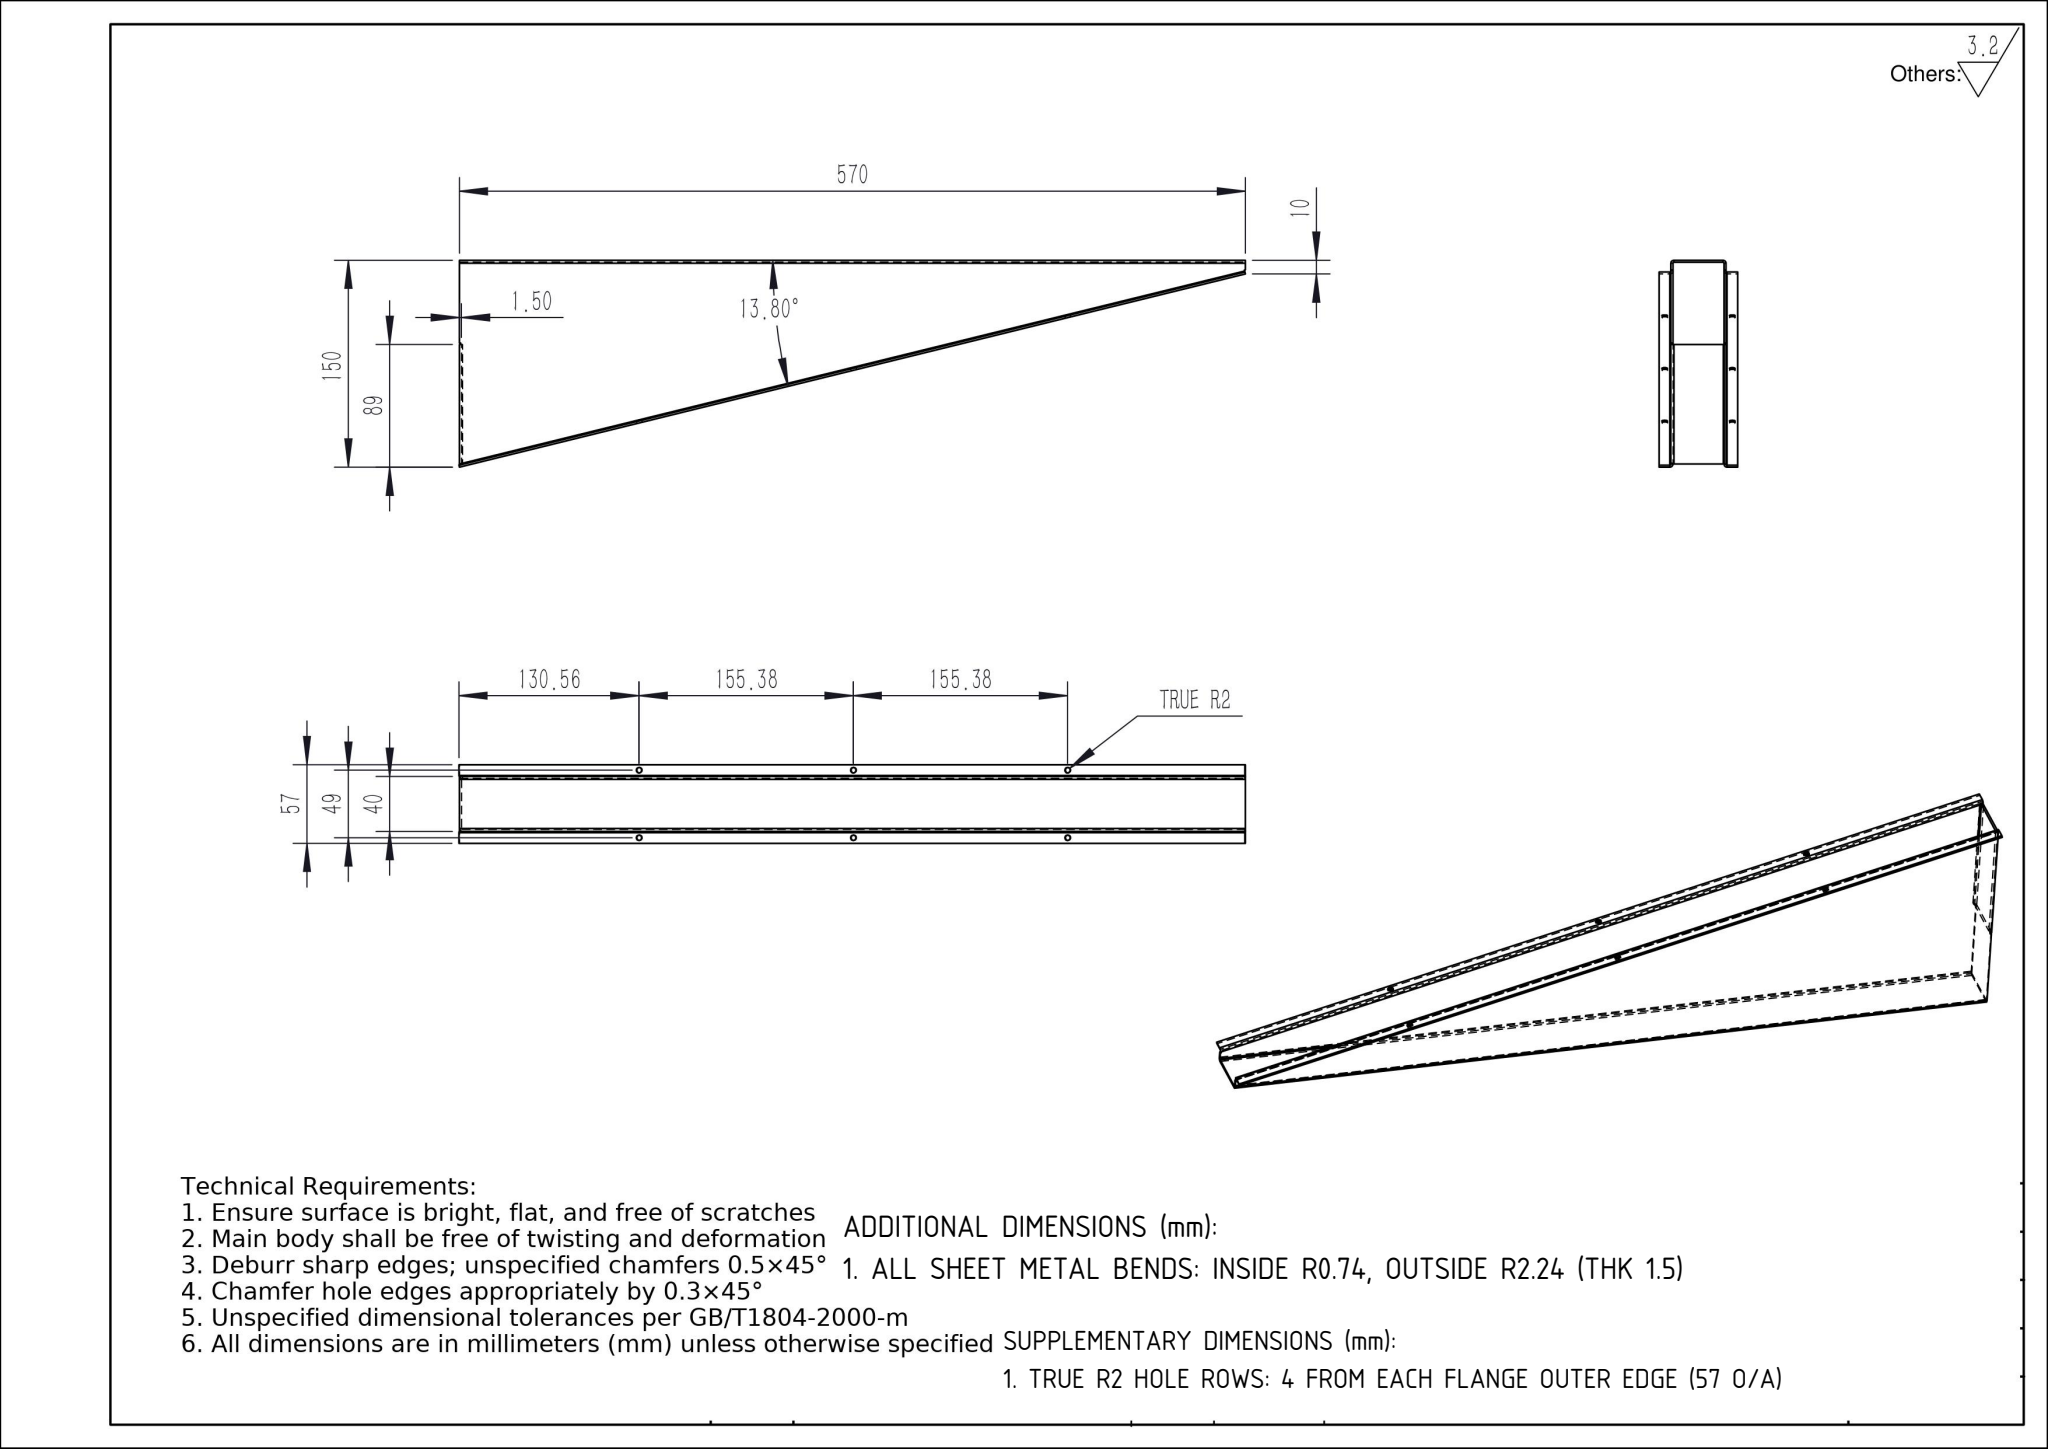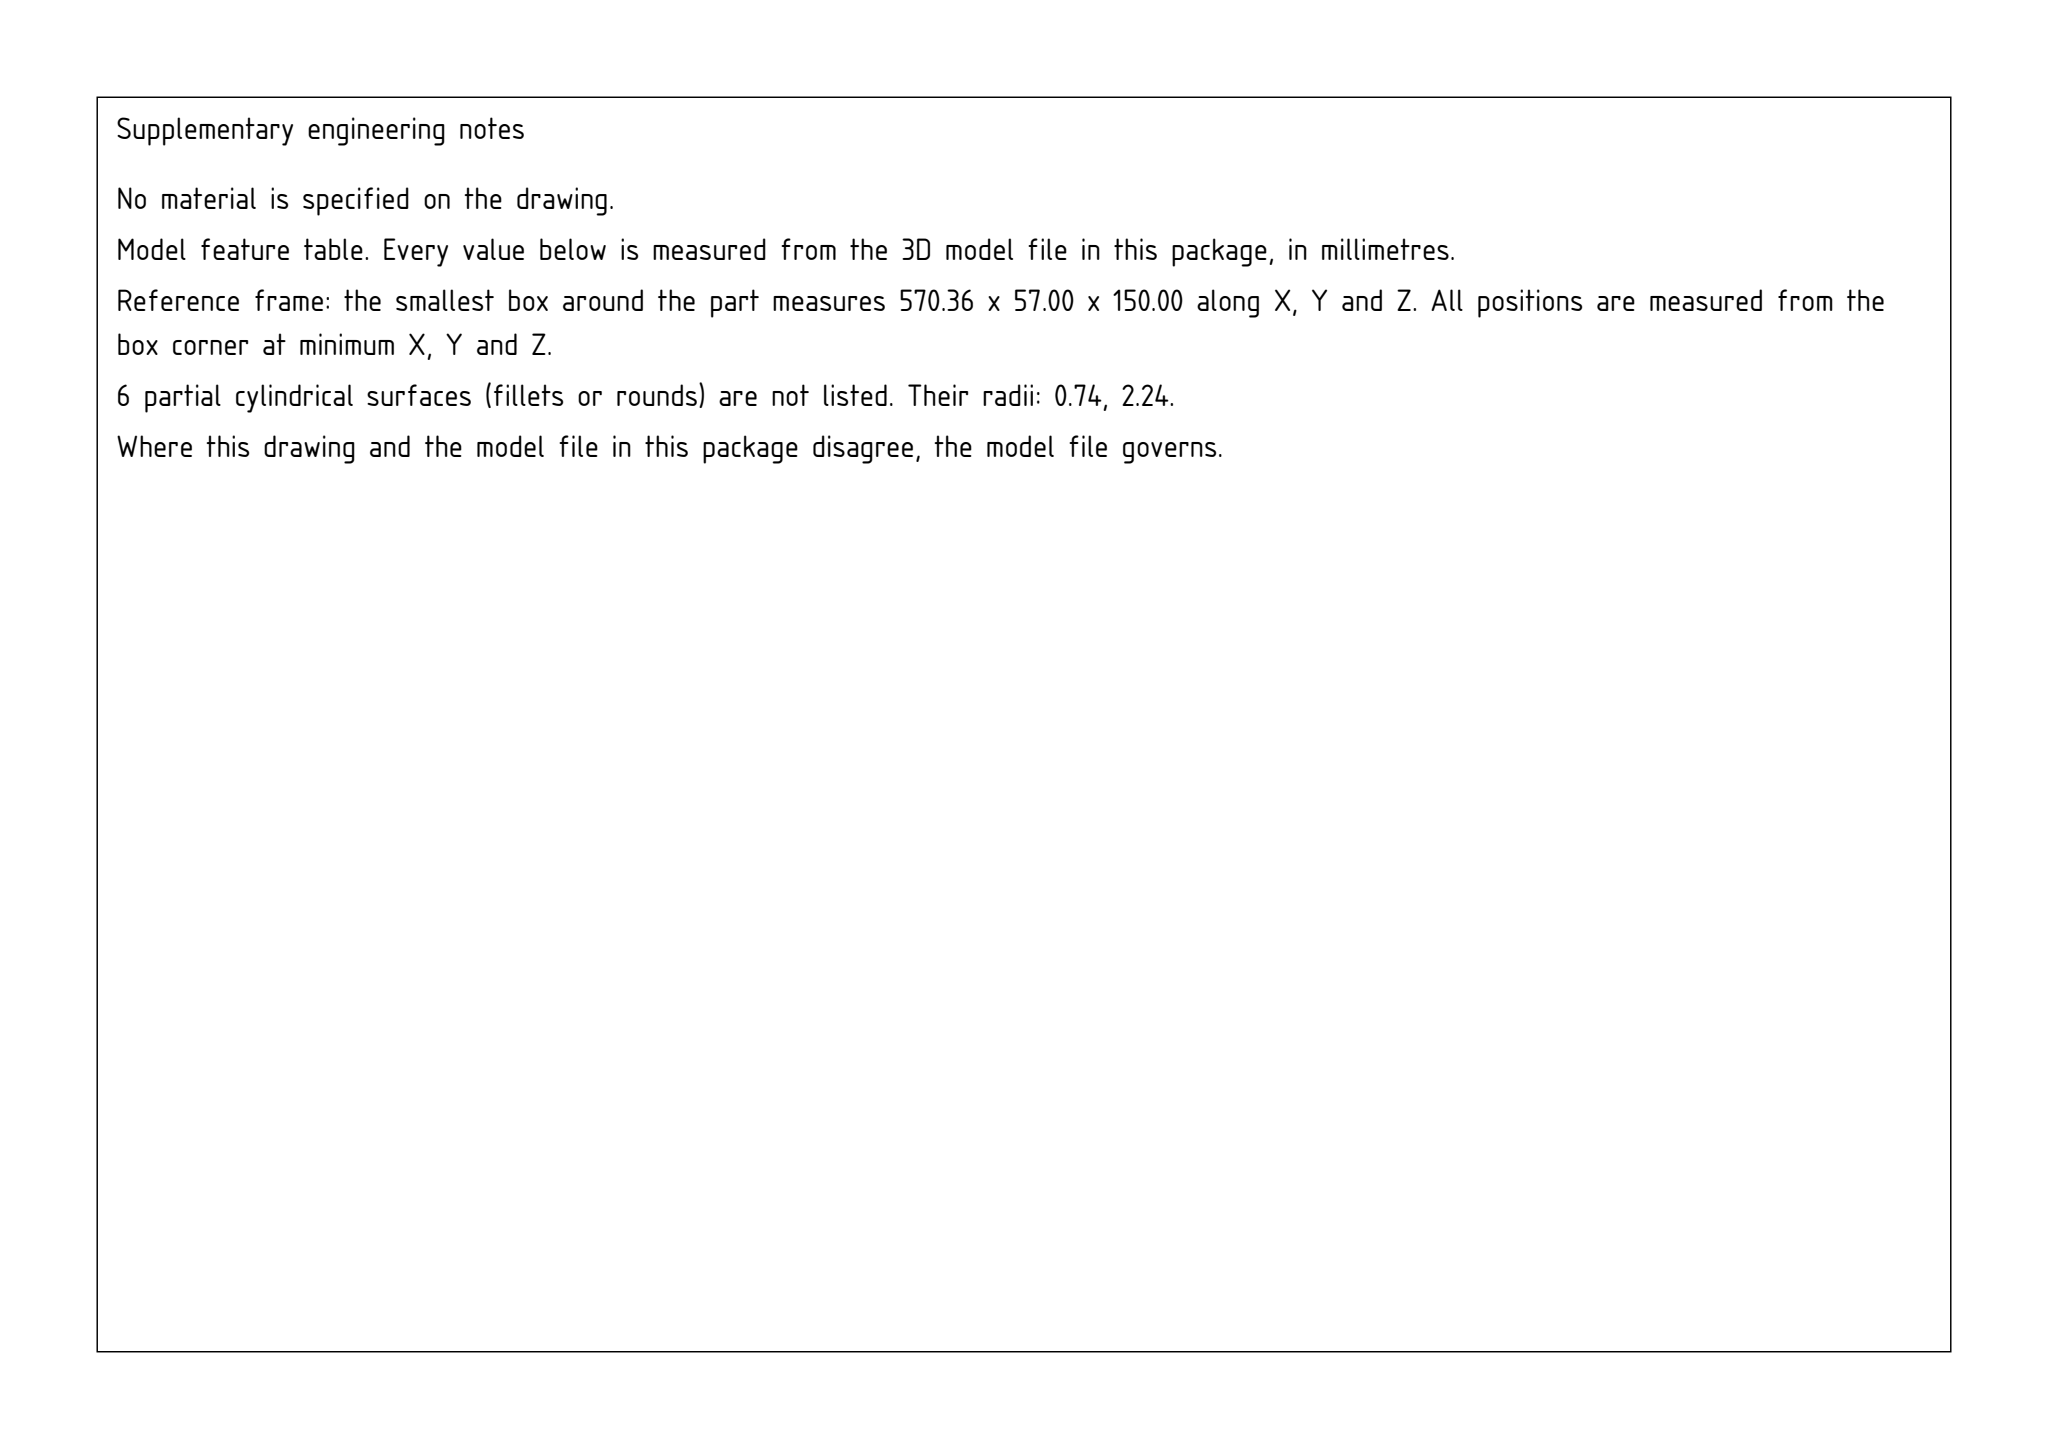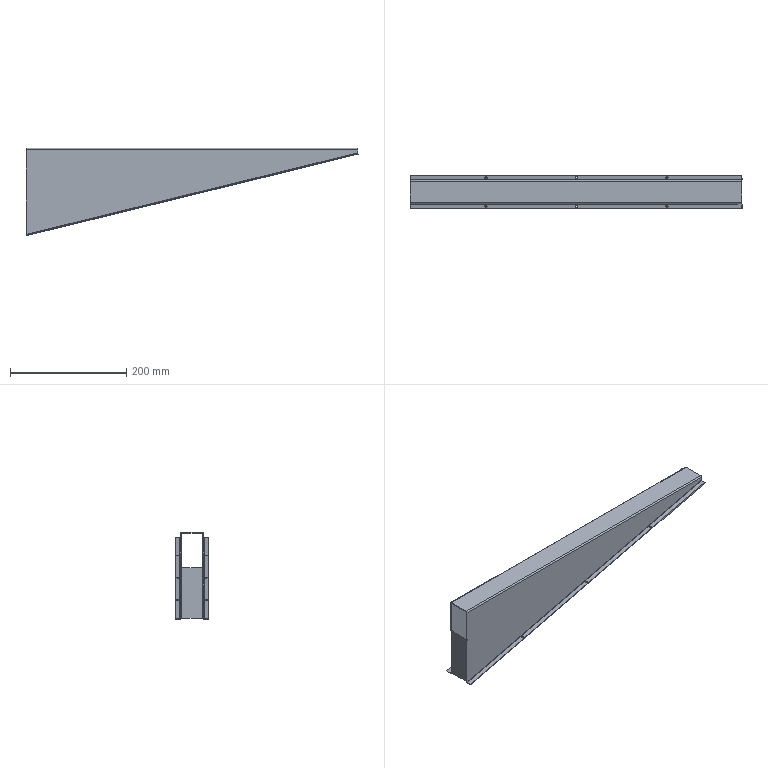Part | SolidWorks | mm | 1 solid | 71 faces | box 570.36 x 57 x 150 mm | volume 185732 mm3 | plane 46 | cylinder 22 | spline 3 | commonest cylinder face diameters 4 x12 4.473 x5 1.473 x5